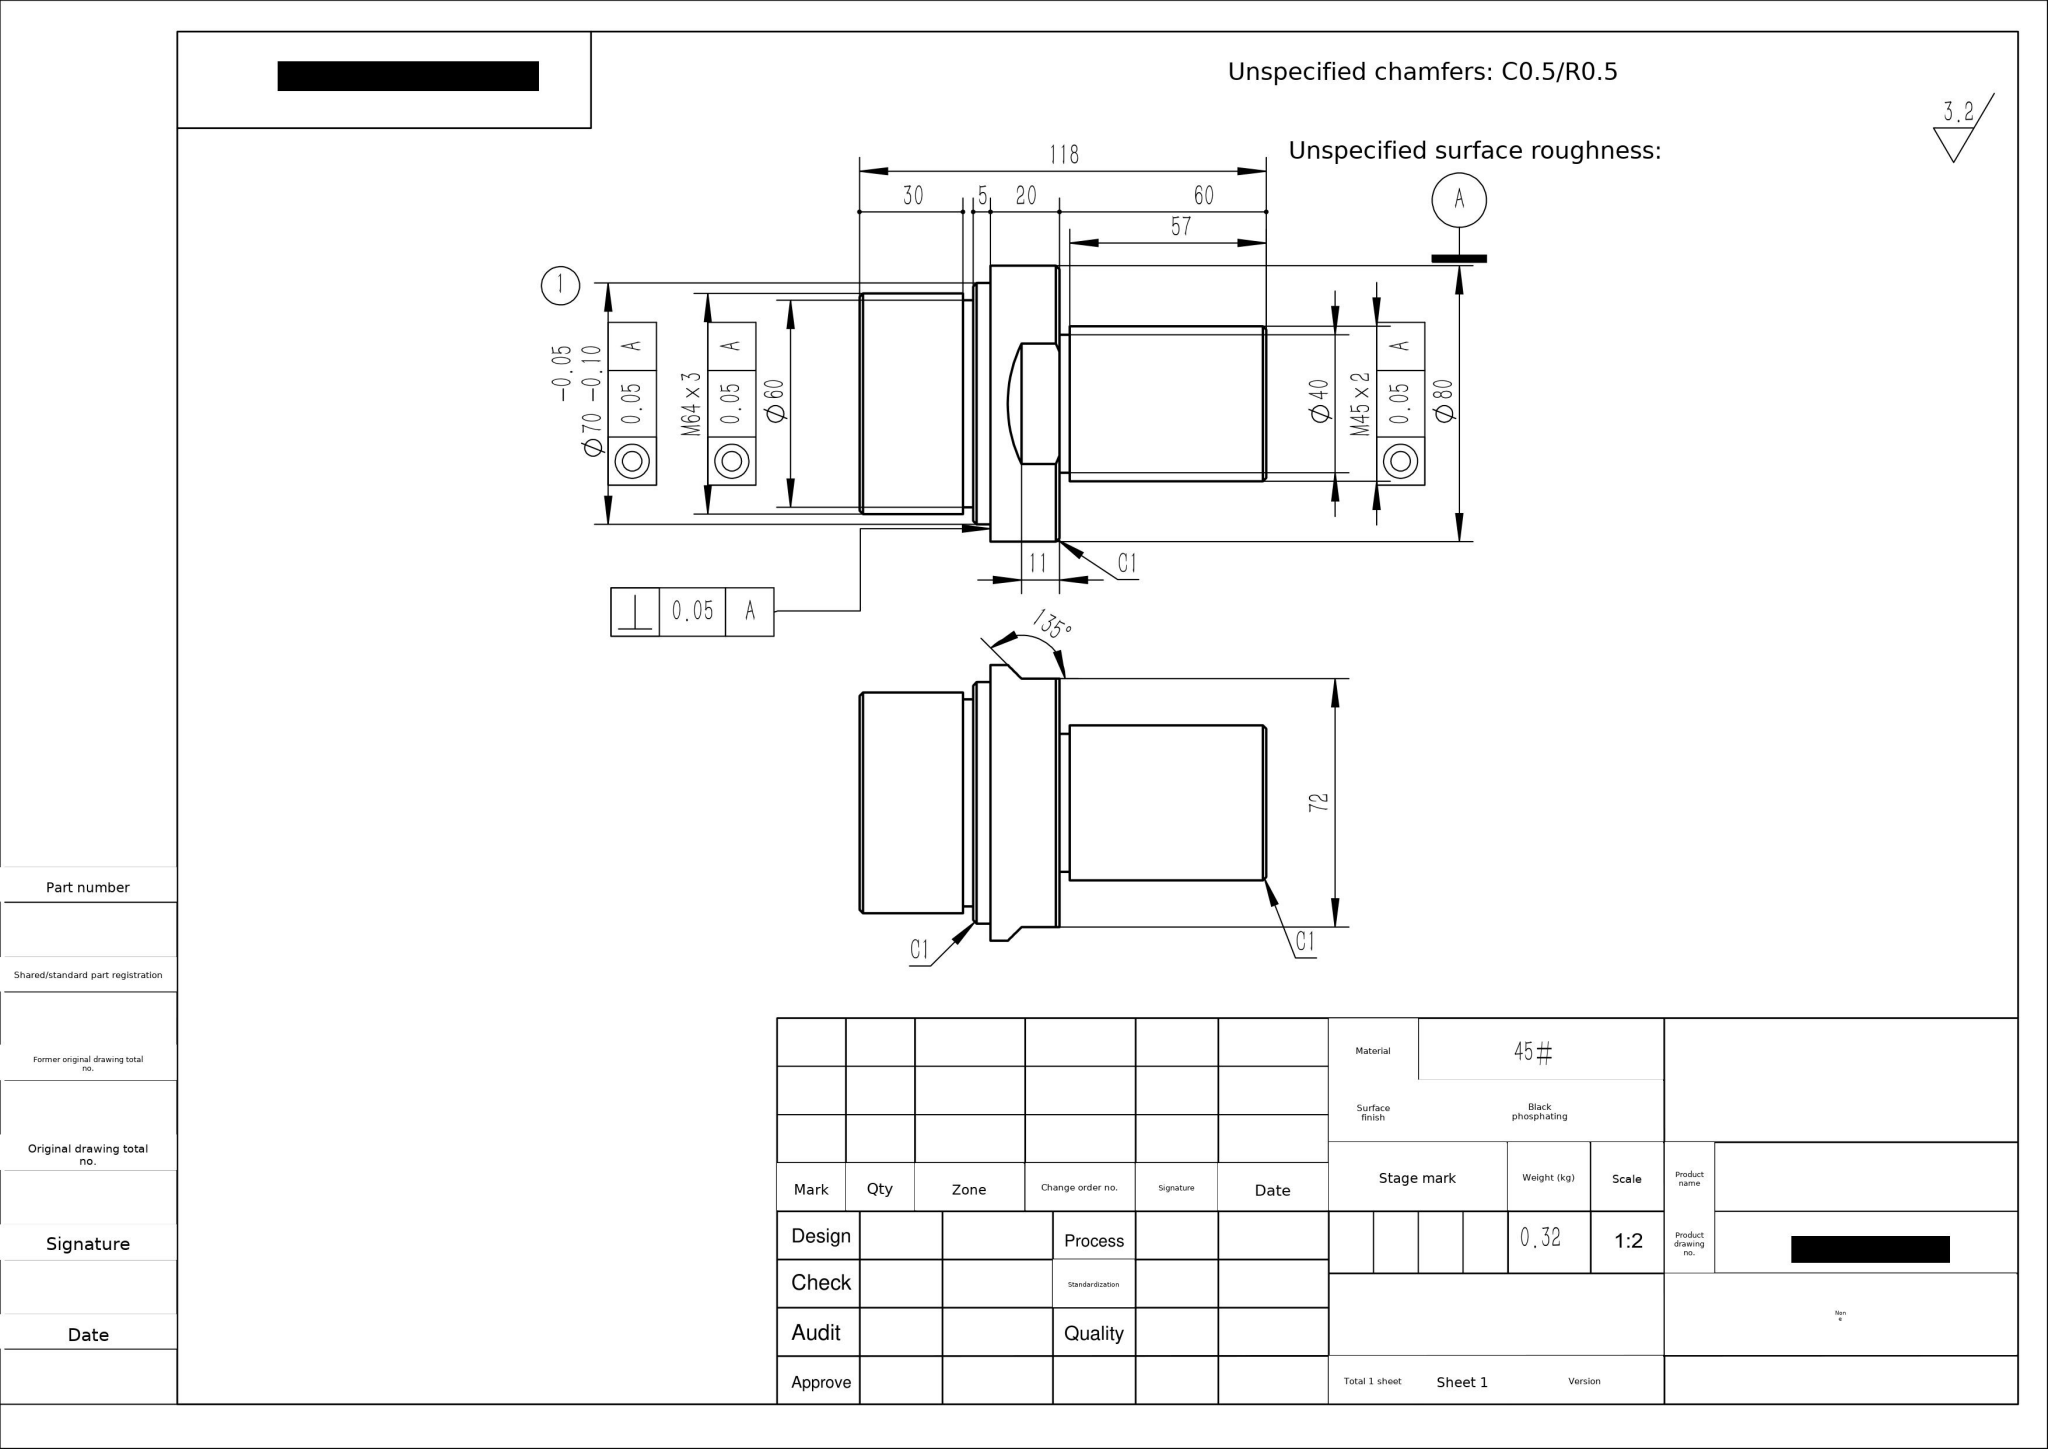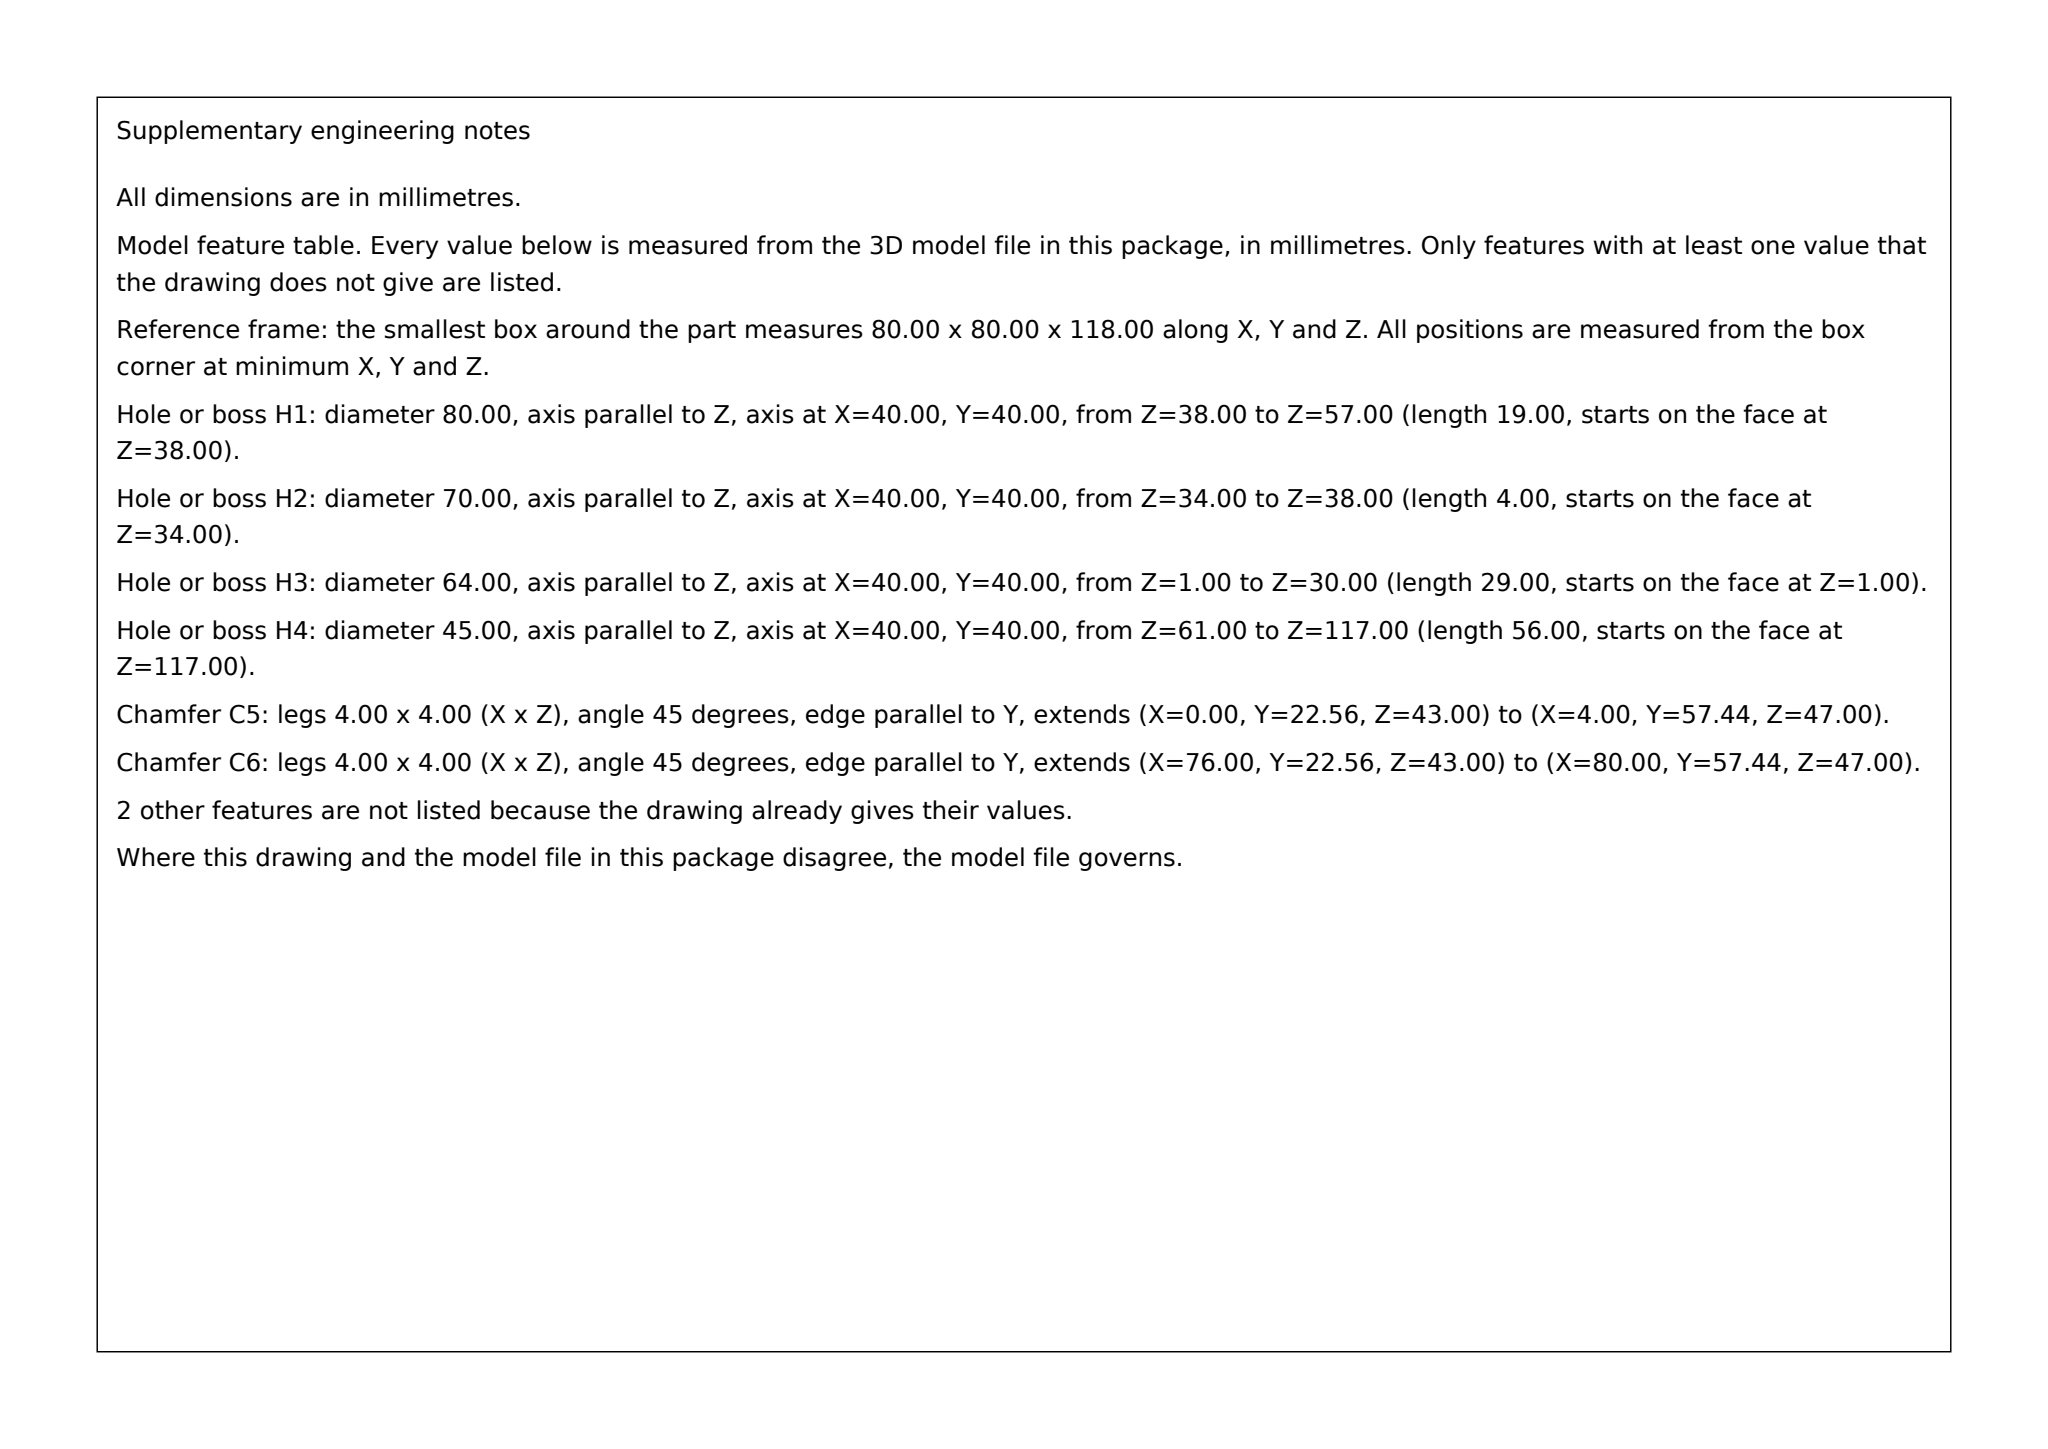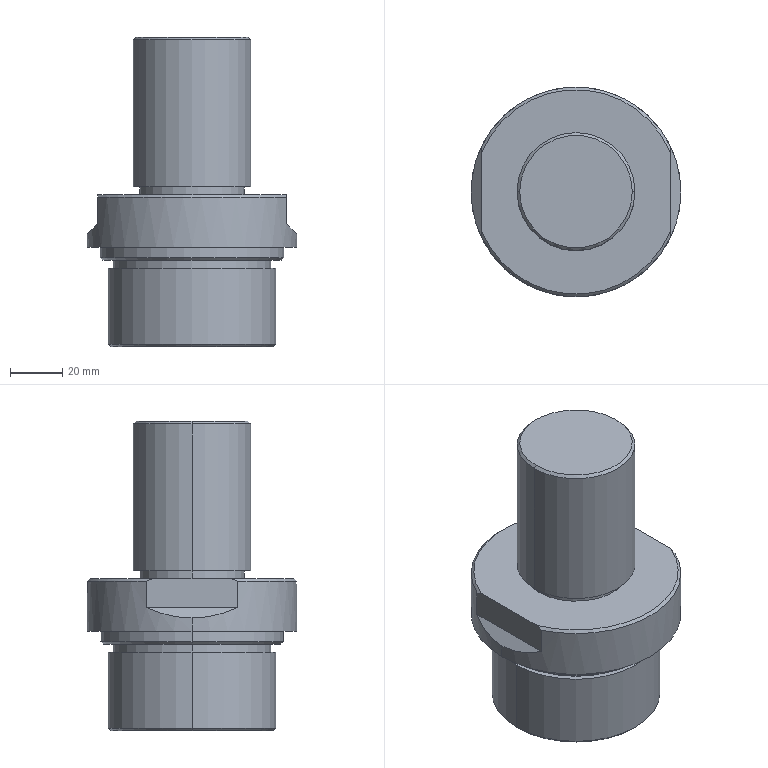Part | SolidWorks | mm | material 45# | 1 solid | 31 faces | box 80 x 80 x 118 mm | volume 316452 mm3 | cylinder 12 | plane 11 | cone 8 | commonest cylinder face diameters 45 x2 40 x2 80 x2 70 x2 60 x2 64 x2
STEP:
#1=CARTESIAN_POINT('',(21.5,0.,118.));
#2=VERTEX_POINT('',#1);
#3=CARTESIAN_POINT('',(-21.5,0.,118.));
#4=VERTEX_POINT('',#3);
#5=CARTESIAN_POINT('',(0.,0.,118.));
#6=DIRECTION('',(0.,0.,1.));
#7=DIRECTION('',(1.,0.,0.));
#8=AXIS2_PLACEMENT_3D('',#5,#6,#7);
#9=CIRCLE('',#8,21.5);
#10=EDGE_CURVE('',#2,#4,#9,.T.);
#11=ORIENTED_EDGE('',*,*,#10,.F.);
#12=CARTESIAN_POINT('',(22.5,0.,117.));
#13=VERTEX_POINT('',#12);
#14=CARTESIAN_POINT('',(21.5,0.,118.));
#15=DIRECTION('',(0.7071,0.,-0.7071));
#16=VECTOR('',#15,1000.);
#17=LINE('',#14,#16);
#18=EDGE_CURVE('',#2,#13,#17,.T.);
#19=ORIENTED_EDGE('',*,*,#18,.T.);
#20=CARTESIAN_POINT('',(-22.5,0.,117.));
#21=VERTEX_POINT('',#20);
#22=CARTESIAN_POINT('',(0.,0.,117.));
#23=DIRECTION('',(0.,0.,-1.));
#24=DIRECTION('',(1.,0.,0.));
#25=AXIS2_PLACEMENT_3D('',#22,#23,#24);
#26=CIRCLE('',#25,22.5);
#27=EDGE_CURVE('',#21,#13,#26,.T.);
#28=ORIENTED_EDGE('',*,*,#27,.F.);
#29=CARTESIAN_POINT('',(-21.5,0.,118.));
#30=DIRECTION('',(-0.7071,0.,-0.7071));
#31=VECTOR('',#30,1000.);
#32=LINE('',#29,#31);
#33=EDGE_CURVE('',#4,#21,#32,.T.);
#34=ORIENTED_EDGE('',*,*,#33,.F.);
#35=EDGE_LOOP('',(#11,#19,#28,#34));
#36=FACE_OUTER_BOUND('',#35,.T.);
#37=CARTESIAN_POINT('',(0.,0.,118.));
#38=DIRECTION('',(0.,0.,-1.));
#39=DIRECTION('',(-1.,0.,0.));
#40=AXIS2_PLACEMENT_3D('',#37,#38,#39);
#41=CONICAL_SURFACE('',#40,21.5,0.7854);
#42=ADVANCED_FACE('',(#36),#41,.T.);
#43=CARTESIAN_POINT('',(-34.,0.,33.));
#44=VERTEX_POINT('',#43);
#45=CARTESIAN_POINT('',(34.,0.,33.));
#46=VERTEX_POINT('',#45);
#47=CARTESIAN_POINT('',(0.,0.,33.));
#48=DIRECTION('',(0.,0.,-1.));
#49=DIRECTION('',(1.,0.,0.));
#50=AXIS2_PLACEMENT_3D('',#47,#48,#49);
#51=CIRCLE('',#50,34.);
#52=EDGE_CURVE('',#44,#46,#51,.T.);
#53=ORIENTED_EDGE('',*,*,#52,.F.);
#54=CARTESIAN_POINT('',(-35.,0.,34.));
#55=VERTEX_POINT('',#54);
#56=CARTESIAN_POINT('',(-35.,0.,34.));
#57=DIRECTION('',(-0.7071,0.,0.7071));
#58=VECTOR('',#57,1000.);
#59=LINE('',#56,#58);
#60=EDGE_CURVE('',#44,#55,#59,.T.);
#61=ORIENTED_EDGE('',*,*,#60,.T.);
#62=CARTESIAN_POINT('',(35.,0.,34.));
#63=VERTEX_POINT('',#62);
#64=CARTESIAN_POINT('',(0.,0.,34.));
#65=DIRECTION('',(0.,0.,1.));
#66=DIRECTION('',(1.,0.,0.));
#67=AXIS2_PLACEMENT_3D('',#64,#65,#66);
#68=CIRCLE('',#67,35.);
#69=EDGE_CURVE('',#63,#55,#68,.T.);
#70=ORIENTED_EDGE('',*,*,#69,.F.);
#71=CARTESIAN_POINT('',(35.,0.,34.));
#72=DIRECTION('',(0.7071,0.,0.7071));
#73=VECTOR('',#72,1000.);
#74=LINE('',#71,#73);
#75=EDGE_CURVE('',#46,#63,#74,.T.);
#76=ORIENTED_EDGE('',*,*,#75,.F.);
#77=EDGE_LOOP('',(#53,#61,#70,#76));
#78=FACE_OUTER_BOUND('',#77,.T.);
#79=CARTESIAN_POINT('',(0.,0.,34.));
#80=DIRECTION('',(0.,0.,1.));
#81=DIRECTION('',(1.,0.,0.));
#82=AXIS2_PLACEMENT_3D('',#79,#80,#81);
#83=CONICAL_SURFACE('',#82,35.,0.7854);
#84=ADVANCED_FACE('',(#78),#83,.T.);
#85=CARTESIAN_POINT('',(-31.,0.,0.));
#86=VERTEX_POINT('',#85);
#87=CARTESIAN_POINT('',(31.,0.,0.));
#88=VERTEX_POINT('',#87);
#89=CARTESIAN_POINT('',(0.,0.,0.));
#90=DIRECTION('',(0.,0.,-1.));
#91=DIRECTION('',(1.,0.,0.));
#92=AXIS2_PLACEMENT_3D('',#89,#90,#91);
#93=CIRCLE('',#92,31.);
#94=EDGE_CURVE('',#86,#88,#93,.T.);
#95=ORIENTED_EDGE('',*,*,#94,.F.);
#96=CARTESIAN_POINT('',(-32.,0.,1.));
#97=VERTEX_POINT('',#96);
#98=CARTESIAN_POINT('',(-32.,0.,1.));
#99=DIRECTION('',(-0.7071,0.,0.7071));
#100=VECTOR('',#99,1000.);
#101=LINE('',#98,#100);
#102=EDGE_CURVE('',#86,#97,#101,.T.);
#103=ORIENTED_EDGE('',*,*,#102,.T.);
#104=CARTESIAN_POINT('',(32.,0.,1.));
#105=VERTEX_POINT('',#104);
#106=CARTESIAN_POINT('',(0.,0.,1.));
#107=DIRECTION('',(0.,0.,1.));
#108=DIRECTION('',(1.,0.,0.));
#109=AXIS2_PLACEMENT_3D('',#106,#107,#108);
#110=CIRCLE('',#109,32.);
#111=EDGE_CURVE('',#105,#97,#110,.T.);
#112=ORIENTED_EDGE('',*,*,#111,.F.);
#113=CARTESIAN_POINT('',(32.,0.,1.));
#114=DIRECTION('',(0.7071,0.,0.7071));
#115=VECTOR('',#114,1000.);
#116=LINE('',#113,#115);
#117=EDGE_CURVE('',#88,#105,#116,.T.);
#118=ORIENTED_EDGE('',*,*,#117,.F.);
#119=EDGE_LOOP('',(#95,#103,#112,#118));
#120=FACE_OUTER_BOUND('',#119,.T.);
#121=CARTESIAN_POINT('',(0.,0.,1.));
#122=DIRECTION('',(0.,0.,1.));
#123=DIRECTION('',(1.,0.,0.));
#124=AXIS2_PLACEMENT_3D('',#121,#122,#123);
#125=CONICAL_SURFACE('',#124,32.,0.7854);
#126=ADVANCED_FACE('',(#120),#125,.T.);
#127=ORIENTED_EDGE('',*,*,#27,.T.);
#128=CARTESIAN_POINT('',(22.5,0.,61.));
#129=VERTEX_POINT('',#128);
#130=CARTESIAN_POINT('',(22.5,0.,118.));
#131=DIRECTION('',(0.,0.,-1.));
#132=VECTOR('',#131,1000.);
#133=LINE('',#130,#132);
#134=EDGE_CURVE('',#13,#129,#133,.T.);
#135=ORIENTED_EDGE('',*,*,#134,.T.);
#136=CARTESIAN_POINT('',(-22.5,0.,61.));
#137=VERTEX_POINT('',#136);
#138=CARTESIAN_POINT('',(0.,0.,61.));
#139=DIRECTION('',(0.,0.,1.));
#140=DIRECTION('',(1.,0.,0.));
#141=AXIS2_PLACEMENT_3D('',#138,#139,#140);
#142=CIRCLE('',#141,22.5);
#143=EDGE_CURVE('',#129,#137,#142,.T.);
#144=ORIENTED_EDGE('',*,*,#143,.T.);
#145=CARTESIAN_POINT('',(-22.5,0.,118.));
#146=DIRECTION('',(0.,0.,-1.));
#147=VECTOR('',#146,1000.);
#148=LINE('',#145,#147);
#149=EDGE_CURVE('',#21,#137,#148,.T.);
#150=ORIENTED_EDGE('',*,*,#149,.F.);
#151=EDGE_LOOP('',(#127,#135,#144,#150));
#152=FACE_OUTER_BOUND('',#151,.T.);
#153=CARTESIAN_POINT('',(0.,0.,118.));
#154=DIRECTION('',(0.,0.,-1.));
#155=DIRECTION('',(-1.,0.,0.));
#156=AXIS2_PLACEMENT_3D('',#153,#154,#155);
#157=CYLINDRICAL_SURFACE('',#156,22.5);
#158=ADVANCED_FACE('',(#152),#157,.T.);
#159=CARTESIAN_POINT('',(20.,0.,61.));
#160=VERTEX_POINT('',#159);
#161=CARTESIAN_POINT('',(-20.,0.,61.));
#162=VERTEX_POINT('',#161);
#163=CARTESIAN_POINT('',(0.,0.,61.));
#164=DIRECTION('',(0.,0.,1.));
#165=DIRECTION('',(1.,0.,0.));
#166=AXIS2_PLACEMENT_3D('',#163,#164,#165);
#167=CIRCLE('',#166,20.);
#168=EDGE_CURVE('',#160,#162,#167,.T.);
#169=ORIENTED_EDGE('',*,*,#168,.F.);
#170=CARTESIAN_POINT('',(20.,0.,58.));
#171=VERTEX_POINT('',#170);
#172=CARTESIAN_POINT('',(20.,0.,61.));
#173=DIRECTION('',(0.,0.,-1.));
#174=VECTOR('',#173,1000.);
#175=LINE('',#172,#174);
#176=EDGE_CURVE('',#160,#171,#175,.T.);
#177=ORIENTED_EDGE('',*,*,#176,.T.);
#178=CARTESIAN_POINT('',(-20.,0.,58.));
#179=VERTEX_POINT('',#178);
#180=CARTESIAN_POINT('',(0.,0.,58.));
#181=DIRECTION('',(0.,0.,1.));
#182=DIRECTION('',(1.,0.,0.));
#183=AXIS2_PLACEMENT_3D('',#180,#181,#182);
#184=CIRCLE('',#183,20.);
#185=EDGE_CURVE('',#171,#179,#184,.T.);
#186=ORIENTED_EDGE('',*,*,#185,.T.);
#187=CARTESIAN_POINT('',(-20.,0.,61.));
#188=DIRECTION('',(0.,0.,-1.));
#189=VECTOR('',#188,1000.);
#190=LINE('',#187,#189);
#191=EDGE_CURVE('',#162,#179,#190,.T.);
#192=ORIENTED_EDGE('',*,*,#191,.F.);
#193=EDGE_LOOP('',(#169,#177,#186,#192));
#194=FACE_OUTER_BOUND('',#193,.T.);
#195=CARTESIAN_POINT('',(0.,0.,61.));
#196=DIRECTION('',(0.,0.,-1.));
#197=DIRECTION('',(-1.,0.,0.));
#198=AXIS2_PLACEMENT_3D('',#195,#196,#197);
#199=CYLINDRICAL_SURFACE('',#198,20.);
#200=ADVANCED_FACE('',(#194),#199,.T.);
#201=CARTESIAN_POINT('',(36.,17.436,47.));
#202=VERTEX_POINT('',#201);
#203=CARTESIAN_POINT('',(40.,0.,43.));
#204=VERTEX_POINT('',#203);
#205=CARTESIAN_POINT('',(36.,17.436,47.));
#206=CARTESIAN_POINT('',(38.644,11.977,44.356));
#207=CARTESIAN_POINT('',(40.,6.065,43.));
#208=CARTESIAN_POINT('',(40.,0.,43.));
#209=(BOUNDED_CURVE()B_SPLINE_CURVE(3,(#205,#206,#207,#208),.UNSPECIFIED.,.F.,.T.)B_SPLINE_CURVE_WITH_KNOTS((4,4),(5.832,6.283),.UNSPECIFIED.)CURVE()GEOMETRIC_REPRESENTATION_ITEM()RATIONAL_B_SPLINE_CURVE((1.,0.9831,0.9831,1.))REPRESENTATION_ITEM(''));
#210=EDGE_CURVE('',#202,#204,#209,.T.);
#211=ORIENTED_EDGE('',*,*,#210,.T.);
#212=CARTESIAN_POINT('',(40.,0.,38.));
#213=VERTEX_POINT('',#212);
#214=CARTESIAN_POINT('',(40.,0.,58.));
#215=DIRECTION('',(0.,0.,-1.));
#216=VECTOR('',#215,1000.);
#217=LINE('',#214,#216);
#218=EDGE_CURVE('',#204,#213,#217,.T.);
#219=ORIENTED_EDGE('',*,*,#218,.T.);
#220=CARTESIAN_POINT('',(-40.,0.,38.));
#221=VERTEX_POINT('',#220);
#222=CARTESIAN_POINT('',(0.,0.,38.));
#223=DIRECTION('',(0.,0.,1.));
#224=DIRECTION('',(1.,0.,0.));
#225=AXIS2_PLACEMENT_3D('',#222,#223,#224);
#226=CIRCLE('',#225,40.);
#227=EDGE_CURVE('',#213,#221,#226,.T.);
#228=ORIENTED_EDGE('',*,*,#227,.T.);
#229=CARTESIAN_POINT('',(-40.,0.,43.));
#230=VERTEX_POINT('',#229);
#231=CARTESIAN_POINT('',(-40.,0.,58.));
#232=DIRECTION('',(0.,0.,-1.));
#233=VECTOR('',#232,1000.);
#234=LINE('',#231,#233);
#235=EDGE_CURVE('',#230,#221,#234,.T.);
#236=ORIENTED_EDGE('',*,*,#235,.F.);
#237=CARTESIAN_POINT('',(-36.,17.436,47.));
#238=VERTEX_POINT('',#237);
#239=CARTESIAN_POINT('',(-40.,0.,43.));
#240=CARTESIAN_POINT('',(-40.,6.065,43.));
#241=CARTESIAN_POINT('',(-38.644,11.977,44.356));
#242=CARTESIAN_POINT('',(-36.,17.436,47.));
#243=(BOUNDED_CURVE()B_SPLINE_CURVE(3,(#239,#240,#241,#242),.UNSPECIFIED.,.F.,.T.)B_SPLINE_CURVE_WITH_KNOTS((4,4),(0.,0.451),.UNSPECIFIED.)CURVE()GEOMETRIC_REPRESENTATION_ITEM()RATIONAL_B_SPLINE_CURVE((1.,0.9831,0.9831,1.))REPRESENTATION_ITEM(''));
#244=EDGE_CURVE('',#230,#238,#243,.T.);
#245=ORIENTED_EDGE('',*,*,#244,.T.);
#246=CARTESIAN_POINT('',(-36.,17.436,57.));
#247=VERTEX_POINT('',#246);
#248=CARTESIAN_POINT('',(-36.,17.436,58.));
#249=DIRECTION('',(0.,0.,1.));
#250=VECTOR('',#249,1000.);
#251=LINE('',#248,#250);
#252=EDGE_CURVE('',#238,#247,#251,.T.);
#253=ORIENTED_EDGE('',*,*,#252,.T.);
#254=CARTESIAN_POINT('',(36.,17.436,57.));
#255=VERTEX_POINT('',#254);
#256=CARTESIAN_POINT('',(0.,0.,57.));
#257=DIRECTION('',(0.,0.,-1.));
#258=DIRECTION('',(1.,0.,0.));
#259=AXIS2_PLACEMENT_3D('',#256,#257,#258);
#260=CIRCLE('',#259,40.);
#261=EDGE_CURVE('',#247,#255,#260,.T.);
#262=ORIENTED_EDGE('',*,*,#261,.T.);
#263=CARTESIAN_POINT('',(36.,17.436,58.));
#264=DIRECTION('',(0.,0.,-1.));
#265=VECTOR('',#264,1000.);
#266=LINE('',#263,#265);
#267=EDGE_CURVE('',#255,#202,#266,.T.);
#268=ORIENTED_EDGE('',*,*,#267,.T.);
#269=EDGE_LOOP('',(#211,#219,#228,#236,#245,#253,#262,#268));
#270=FACE_OUTER_BOUND('',#269,.T.);
#271=CARTESIAN_POINT('',(0.,0.,58.));
#272=DIRECTION('',(0.,0.,-1.));
#273=DIRECTION('',(-1.,0.,0.));
#274=AXIS2_PLACEMENT_3D('',#271,#272,#273);
#275=CYLINDRICAL_SURFACE('',#274,40.);
#276=ADVANCED_FACE('',(#270),#275,.T.);
#277=CARTESIAN_POINT('',(35.,0.,38.));
#278=VERTEX_POINT('',#277);
#279=CARTESIAN_POINT('',(-35.,0.,38.));
#280=VERTEX_POINT('',#279);
#281=CARTESIAN_POINT('',(0.,0.,38.));
#282=DIRECTION('',(0.,0.,1.));
#283=DIRECTION('',(1.,0.,0.));
#284=AXIS2_PLACEMENT_3D('',#281,#282,#283);
#285=CIRCLE('',#284,35.);
#286=EDGE_CURVE('',#278,#280,#285,.T.);
#287=ORIENTED_EDGE('',*,*,#286,.F.);
#288=CARTESIAN_POINT('',(35.,0.,38.));
#289=DIRECTION('',(0.,0.,-1.));
#290=VECTOR('',#289,1000.);
#291=LINE('',#288,#290);
#292=EDGE_CURVE('',#278,#63,#291,.T.);
#293=ORIENTED_EDGE('',*,*,#292,.T.);
#294=ORIENTED_EDGE('',*,*,#69,.T.);
#295=CARTESIAN_POINT('',(-35.,0.,38.));
#296=DIRECTION('',(0.,0.,-1.));
#297=VECTOR('',#296,1000.);
#298=LINE('',#295,#297);
#299=EDGE_CURVE('',#280,#55,#298,.T.);
#300=ORIENTED_EDGE('',*,*,#299,.F.);
#301=EDGE_LOOP('',(#287,#293,#294,#300));
#302=FACE_OUTER_BOUND('',#301,.T.);
#303=CARTESIAN_POINT('',(0.,0.,38.));
#304=DIRECTION('',(0.,0.,-1.));
#305=DIRECTION('',(-1.,0.,0.));
#306=AXIS2_PLACEMENT_3D('',#303,#304,#305);
#307=CYLINDRICAL_SURFACE('',#306,35.);
#308=ADVANCED_FACE('',(#302),#307,.T.);
#309=CARTESIAN_POINT('',(30.,0.,33.));
#310=VERTEX_POINT('',#309);
#311=CARTESIAN_POINT('',(-30.,0.,33.));
#312=VERTEX_POINT('',#311);
#313=CARTESIAN_POINT('',(0.,0.,33.));
#314=DIRECTION('',(0.,0.,1.));
#315=DIRECTION('',(1.,0.,0.));
#316=AXIS2_PLACEMENT_3D('',#313,#314,#315);
#317=CIRCLE('',#316,30.);
#318=EDGE_CURVE('',#310,#312,#317,.T.);
#319=ORIENTED_EDGE('',*,*,#318,.F.);
#320=CARTESIAN_POINT('',(30.,0.,30.));
#321=VERTEX_POINT('',#320);
#322=CARTESIAN_POINT('',(30.,0.,33.));
#323=DIRECTION('',(0.,0.,-1.));
#324=VECTOR('',#323,1000.);
#325=LINE('',#322,#324);
#326=EDGE_CURVE('',#310,#321,#325,.T.);
#327=ORIENTED_EDGE('',*,*,#326,.T.);
#328=CARTESIAN_POINT('',(-30.,0.,30.));
#329=VERTEX_POINT('',#328);
#330=CARTESIAN_POINT('',(0.,0.,30.));
#331=DIRECTION('',(0.,0.,1.));
#332=DIRECTION('',(1.,0.,0.));
#333=AXIS2_PLACEMENT_3D('',#330,#331,#332);
#334=CIRCLE('',#333,30.);
#335=EDGE_CURVE('',#321,#329,#334,.T.);
#336=ORIENTED_EDGE('',*,*,#335,.T.);
#337=CARTESIAN_POINT('',(-30.,0.,33.));
#338=DIRECTION('',(0.,0.,-1.));
#339=VECTOR('',#338,1000.);
#340=LINE('',#337,#339);
#341=EDGE_CURVE('',#312,#329,#340,.T.);
#342=ORIENTED_EDGE('',*,*,#341,.F.);
#343=EDGE_LOOP('',(#319,#327,#336,#342));
#344=FACE_OUTER_BOUND('',#343,.T.);
#345=CARTESIAN_POINT('',(0.,0.,33.));
#346=DIRECTION('',(0.,0.,-1.));
#347=DIRECTION('',(-1.,0.,0.));
#348=AXIS2_PLACEMENT_3D('',#345,#346,#347);
#349=CYLINDRICAL_SURFACE('',#348,30.);
#350=ADVANCED_FACE('',(#344),#349,.T.);
#351=CARTESIAN_POINT('',(32.,0.,30.));
#352=VERTEX_POINT('',#351);
#353=CARTESIAN_POINT('',(-32.,0.,30.));
#354=VERTEX_POINT('',#353);
#355=CARTESIAN_POINT('',(0.,0.,30.));
#356=DIRECTION('',(0.,0.,1.));
#357=DIRECTION('',(1.,0.,0.));
#358=AXIS2_PLACEMENT_3D('',#355,#356,#357);
#359=CIRCLE('',#358,32.);
#360=EDGE_CURVE('',#352,#354,#359,.T.);
#361=ORIENTED_EDGE('',*,*,#360,.F.);
#362=CARTESIAN_POINT('',(32.,0.,30.));
#363=DIRECTION('',(0.,0.,-1.));
#364=VECTOR('',#363,1000.);
#365=LINE('',#362,#364);
#366=EDGE_CURVE('',#352,#105,#365,.T.);
#367=ORIENTED_EDGE('',*,*,#366,.T.);
#368=ORIENTED_EDGE('',*,*,#111,.T.);
#369=CARTESIAN_POINT('',(-32.,0.,30.));
#370=DIRECTION('',(0.,0.,-1.));
#371=VECTOR('',#370,1000.);
#372=LINE('',#369,#371);
#373=EDGE_CURVE('',#354,#97,#372,.T.);
#374=ORIENTED_EDGE('',*,*,#373,.F.);
#375=EDGE_LOOP('',(#361,#367,#368,#374));
#376=FACE_OUTER_BOUND('',#375,.T.);
#377=CARTESIAN_POINT('',(0.,0.,30.));
#378=DIRECTION('',(0.,0.,-1.));
#379=DIRECTION('',(-1.,0.,0.));
#380=AXIS2_PLACEMENT_3D('',#377,#378,#379);
#381=CYLINDRICAL_SURFACE('',#380,32.);
#382=ADVANCED_FACE('',(#376),#381,.T.);
#383=CARTESIAN_POINT('',(-36.,-17.436,57.));
#384=VERTEX_POINT('',#383);
#385=CARTESIAN_POINT('',(-36.,-15.,58.));
#386=VERTEX_POINT('',#385);
#387=CARTESIAN_POINT('',(-36.,-17.436,57.));
#388=CARTESIAN_POINT('',(-36.,-16.631,57.351));
#389=CARTESIAN_POINT('',(-36.,-15.82,57.685));
#390=CARTESIAN_POINT('',(-36.,-15.,58.));
#391=B_SPLINE_CURVE_WITH_KNOTS('',3,(#387,#388,#389,#390),.UNSPECIFIED.,.F.,.F.,(4,4),(0.07863,0.08127),.UNSPECIFIED.);
#392=EDGE_CURVE('',#384,#386,#391,.T.);
#393=ORIENTED_EDGE('',*,*,#392,.F.);
#394=CARTESIAN_POINT('',(36.,-17.436,57.));
#395=VERTEX_POINT('',#394);
#396=CARTESIAN_POINT('',(0.,0.,57.));
#397=DIRECTION('',(0.,0.,-1.));
#398=DIRECTION('',(1.,0.,0.));
#399=AXIS2_PLACEMENT_3D('',#396,#397,#398);
#400=CIRCLE('',#399,40.);
#401=EDGE_CURVE('',#395,#384,#400,.T.);
#402=ORIENTED_EDGE('',*,*,#401,.F.);
#403=CARTESIAN_POINT('',(36.,-15.,58.));
#404=VERTEX_POINT('',#403);
#405=CARTESIAN_POINT('',(36.,-15.,58.));
#406=CARTESIAN_POINT('',(36.,-15.822,57.684));
#407=CARTESIAN_POINT('',(36.,-16.634,57.35));
#408=CARTESIAN_POINT('',(36.,-17.436,57.));
#409=B_SPLINE_CURVE_WITH_KNOTS('',3,(#405,#406,#407,#408),.UNSPECIFIED.,.F.,.F.,(4,4),(0.112,0.1146),.UNSPECIFIED.);
#410=EDGE_CURVE('',#404,#395,#409,.T.);
#411=ORIENTED_EDGE('',*,*,#410,.F.);
#412=CARTESIAN_POINT('',(0.,0.,58.));
#413=DIRECTION('',(0.,0.,1.));
#414=DIRECTION('',(1.,0.,0.));
#415=AXIS2_PLACEMENT_3D('',#412,#413,#414);
#416=CIRCLE('',#415,39.);
#417=EDGE_CURVE('',#386,#404,#416,.T.);
#418=ORIENTED_EDGE('',*,*,#417,.F.);
#419=EDGE_LOOP('',(#393,#402,#411,#418));
#420=FACE_OUTER_BOUND('',#419,.T.);
#421=CARTESIAN_POINT('',(0.,0.,58.));
#422=DIRECTION('',(0.,0.,-1.));
#423=DIRECTION('',(-1.,0.,0.));
#424=AXIS2_PLACEMENT_3D('',#421,#422,#423);
#425=CONICAL_SURFACE('',#424,39.,0.7854);
#426=ADVANCED_FACE('',(#420),#425,.T.);
#427=ORIENTED_EDGE('',*,*,#366,.F.);
#428=CARTESIAN_POINT('',(0.,0.,30.));
#429=DIRECTION('',(0.,0.,1.));
#430=DIRECTION('',(1.,0.,0.));
#431=AXIS2_PLACEMENT_3D('',#428,#429,#430);
#432=CIRCLE('',#431,32.);
#433=EDGE_CURVE('',#354,#352,#432,.T.);
#434=ORIENTED_EDGE('',*,*,#433,.F.);
#435=ORIENTED_EDGE('',*,*,#373,.T.);
#436=CARTESIAN_POINT('',(0.,0.,1.));
#437=DIRECTION('',(0.,0.,1.));
#438=DIRECTION('',(1.,0.,0.));
#439=AXIS2_PLACEMENT_3D('',#436,#437,#438);
#440=CIRCLE('',#439,32.);
#441=EDGE_CURVE('',#97,#105,#440,.T.);
#442=ORIENTED_EDGE('',*,*,#441,.T.);
#443=EDGE_LOOP('',(#427,#434,#435,#442));
#444=FACE_OUTER_BOUND('',#443,.T.);
#445=CARTESIAN_POINT('',(0.,0.,30.));
#446=DIRECTION('',(0.,0.,-1.));
#447=DIRECTION('',(-1.,0.,0.));
#448=AXIS2_PLACEMENT_3D('',#445,#446,#447);
#449=CYLINDRICAL_SURFACE('',#448,32.);
#450=ADVANCED_FACE('',(#444),#449,.T.);
#451=CARTESIAN_POINT('',(0.,0.,30.));
#452=DIRECTION('',(0.,0.,1.));
#453=DIRECTION('',(1.,0.,0.));
#454=AXIS2_PLACEMENT_3D('',#451,#452,#453);
#455=CIRCLE('',#454,30.);
#456=EDGE_CURVE('',#329,#321,#455,.T.);
#457=ORIENTED_EDGE('',*,*,#456,.F.);
#458=ORIENTED_EDGE('',*,*,#335,.F.);
#459=EDGE_LOOP('',(#457,#458));
#460=FACE_BOUND('',#459,.T.);
#461=ORIENTED_EDGE('',*,*,#433,.T.);
#462=ORIENTED_EDGE('',*,*,#360,.T.);
#463=EDGE_LOOP('',(#461,#462));
#464=FACE_OUTER_BOUND('',#463,.T.);
#465=CARTESIAN_POINT('',(0.,0.,30.));
#466=DIRECTION('',(0.,0.,1.));
#467=DIRECTION('',(1.,0.,0.));
#468=AXIS2_PLACEMENT_3D('',#465,#466,#467);
#469=PLANE('',#468);
#470=ADVANCED_FACE('',(#460,#464),#469,.T.);
#471=CARTESIAN_POINT('',(0.,0.,0.));
#472=DIRECTION('',(0.,0.,-1.));
#473=DIRECTION('',(1.,0.,0.));
#474=AXIS2_PLACEMENT_3D('',#471,#472,#473);
#475=CIRCLE('',#474,31.);
#476=EDGE_CURVE('',#88,#86,#475,.T.);
#477=ORIENTED_EDGE('',*,*,#476,.T.);
#478=ORIENTED_EDGE('',*,*,#94,.T.);
#479=EDGE_LOOP('',(#477,#478));
#480=FACE_OUTER_BOUND('',#479,.T.);
#481=CARTESIAN_POINT('',(0.,0.,0.));
#482=DIRECTION('',(0.,0.,1.));
#483=DIRECTION('',(1.,0.,0.));
#484=AXIS2_PLACEMENT_3D('',#481,#482,#483);
#485=PLANE('',#484);
#486=ADVANCED_FACE('',(#480),#485,.F.);
#487=ORIENTED_EDGE('',*,*,#326,.F.);
#488=CARTESIAN_POINT('',(0.,0.,33.));
#489=DIRECTION('',(0.,0.,1.));
#490=DIRECTION('',(1.,0.,0.));
#491=AXIS2_PLACEMENT_3D('',#488,#489,#490);
#492=CIRCLE('',#491,30.);
#493=EDGE_CURVE('',#312,#310,#492,.T.);
#494=ORIENTED_EDGE('',*,*,#493,.F.);
#495=ORIENTED_EDGE('',*,*,#341,.T.);
#496=ORIENTED_EDGE('',*,*,#456,.T.);
#497=EDGE_LOOP('',(#487,#494,#495,#496));
#498=FACE_OUTER_BOUND('',#497,.T.);
#499=CARTESIAN_POINT('',(0.,0.,33.));
#500=DIRECTION('',(0.,0.,-1.));
#501=DIRECTION('',(-1.,0.,0.));
#502=AXIS2_PLACEMENT_3D('',#499,#500,#501);
#503=CYLINDRICAL_SURFACE('',#502,30.);
#504=ADVANCED_FACE('',(#498),#503,.T.);
#505=ORIENTED_EDGE('',*,*,#292,.F.);
#506=CARTESIAN_POINT('',(0.,0.,38.));
#507=DIRECTION('',(0.,0.,1.));
#508=DIRECTION('',(1.,0.,0.));
#509=AXIS2_PLACEMENT_3D('',#506,#507,#508);
#510=CIRCLE('',#509,35.);
#511=EDGE_CURVE('',#280,#278,#510,.T.);
#512=ORIENTED_EDGE('',*,*,#511,.F.);
#513=ORIENTED_EDGE('',*,*,#299,.T.);
#514=CARTESIAN_POINT('',(0.,0.,34.));
#515=DIRECTION('',(0.,0.,1.));
#516=DIRECTION('',(1.,0.,0.));
#517=AXIS2_PLACEMENT_3D('',#514,#515,#516);
#518=CIRCLE('',#517,35.);
#519=EDGE_CURVE('',#55,#63,#518,.T.);
#520=ORIENTED_EDGE('',*,*,#519,.T.);
#521=EDGE_LOOP('',(#505,#512,#513,#520));
#522=FACE_OUTER_BOUND('',#521,.T.);
#523=CARTESIAN_POINT('',(0.,0.,38.));
#524=DIRECTION('',(0.,0.,-1.));
#525=DIRECTION('',(-1.,0.,0.));
#526=AXIS2_PLACEMENT_3D('',#523,#524,#525);
#527=CYLINDRICAL_SURFACE('',#526,35.);
#528=ADVANCED_FACE('',(#522),#527,.T.);
#529=CARTESIAN_POINT('',(0.,0.,33.));
#530=DIRECTION('',(0.,0.,-1.));
#531=DIRECTION('',(1.,0.,0.));
#532=AXIS2_PLACEMENT_3D('',#529,#530,#531);
#533=CIRCLE('',#532,34.);
#534=EDGE_CURVE('',#46,#44,#533,.T.);
#535=ORIENTED_EDGE('',*,*,#534,.T.);
#536=ORIENTED_EDGE('',*,*,#52,.T.);
#537=EDGE_LOOP('',(#535,#536));
#538=FACE_OUTER_BOUND('',#537,.T.);
#539=ORIENTED_EDGE('',*,*,#493,.T.);
#540=ORIENTED_EDGE('',*,*,#318,.T.);
#541=EDGE_LOOP('',(#539,#540));
#542=FACE_BOUND('',#541,.T.);
#543=CARTESIAN_POINT('',(0.,0.,33.));
#544=DIRECTION('',(0.,0.,1.));
#545=DIRECTION('',(1.,0.,0.));
#546=AXIS2_PLACEMENT_3D('',#543,#544,#545);
#547=PLANE('',#546);
#548=ADVANCED_FACE('',(#538,#542),#547,.F.);
#549=ORIENTED_EDGE('',*,*,#218,.F.);
#550=CARTESIAN_POINT('',(36.,-17.436,47.));
#551=VERTEX_POINT('',#550);
#552=CARTESIAN_POINT('',(40.,0.,43.));
#553=CARTESIAN_POINT('',(40.,-6.065,43.));
#554=CARTESIAN_POINT('',(38.644,-11.977,44.356));
#555=CARTESIAN_POINT('',(36.,-17.436,47.));
#556=(BOUNDED_CURVE()B_SPLINE_CURVE(3,(#552,#553,#554,#555),.UNSPECIFIED.,.F.,.T.)B_SPLINE_CURVE_WITH_KNOTS((4,4),(0.,0.451),.UNSPECIFIED.)CURVE()GEOMETRIC_REPRESENTATION_ITEM()RATIONAL_B_SPLINE_CURVE((1.,0.9831,0.9831,1.))REPRESENTATION_ITEM(''));
#557=EDGE_CURVE('',#204,#551,#556,.T.);
#558=ORIENTED_EDGE('',*,*,#557,.T.);
#559=CARTESIAN_POINT('',(36.,-17.436,58.));
#560=DIRECTION('',(0.,0.,1.));
#561=VECTOR('',#560,1000.);
#562=LINE('',#559,#561);
#563=EDGE_CURVE('',#551,#395,#562,.T.);
#564=ORIENTED_EDGE('',*,*,#563,.T.);
#565=ORIENTED_EDGE('',*,*,#401,.T.);
#566=CARTESIAN_POINT('',(-36.,-17.436,47.));
#567=VERTEX_POINT('',#566);
#568=CARTESIAN_POINT('',(-36.,-17.436,58.));
#569=DIRECTION('',(0.,0.,-1.));
#570=VECTOR('',#569,1000.);
#571=LINE('',#568,#570);
#572=EDGE_CURVE('',#384,#567,#571,.T.);
#573=ORIENTED_EDGE('',*,*,#572,.T.);
#574=CARTESIAN_POINT('',(-36.,-17.436,47.));
#575=CARTESIAN_POINT('',(-38.644,-11.977,44.356));
#576=CARTESIAN_POINT('',(-40.,-6.065,43.));
#577=CARTESIAN_POINT('',(-40.,0.,43.));
#578=(BOUNDED_CURVE()B_SPLINE_CURVE(3,(#574,#575,#576,#577),.UNSPECIFIED.,.F.,.T.)B_SPLINE_CURVE_WITH_KNOTS((4,4),(5.832,6.283),.UNSPECIFIED.)CURVE()GEOMETRIC_REPRESENTATION_ITEM()RATIONAL_B_SPLINE_CURVE((1.,0.9831,0.9831,1.))REPRESENTATION_ITEM(''));
#579=EDGE_CURVE('',#567,#230,#578,.T.);
#580=ORIENTED_EDGE('',*,*,#579,.T.);
#581=ORIENTED_EDGE('',*,*,#235,.T.);
#582=CARTESIAN_POINT('',(0.,0.,38.));
#583=DIRECTION('',(0.,0.,1.));
#584=DIRECTION('',(1.,0.,0.));
#585=AXIS2_PLACEMENT_3D('',#582,#583,#584);
#586=CIRCLE('',#585,40.);
#587=EDGE_CURVE('',#221,#213,#586,.T.);
#588=ORIENTED_EDGE('',*,*,#587,.T.);
#589=EDGE_LOOP('',(#549,#558,#564,#565,#573,#580,#581,#588));
#590=FACE_OUTER_BOUND('',#589,.T.);
#591=CARTESIAN_POINT('',(0.,0.,58.));
#592=DIRECTION('',(0.,0.,-1.));
#593=DIRECTION('',(-1.,0.,0.));
#594=AXIS2_PLACEMENT_3D('',#591,#592,#593);
#595=CYLINDRICAL_SURFACE('',#594,40.);
#596=ADVANCED_FACE('',(#590),#595,.T.);
#597=CARTESIAN_POINT('',(-36.,15.,58.));
#598=VERTEX_POINT('',#597);
#599=CARTESIAN_POINT('',(-36.,56.293,58.));
#600=DIRECTION('',(-0.,1.,0.));
#601=VECTOR('',#600,1000.);
#602=LINE('',#599,#601);
#603=EDGE_CURVE('',#386,#598,#602,.T.);
#604=ORIENTED_EDGE('',*,*,#603,.F.);
#605=ORIENTED_EDGE('',*,*,#417,.T.);
#606=CARTESIAN_POINT('',(36.,15.,58.));
#607=VERTEX_POINT('',#606);
#608=CARTESIAN_POINT('',(36.,56.293,58.));
#609=DIRECTION('',(-0.,-1.,0.));
#610=VECTOR('',#609,1000.);
#611=LINE('',#608,#610);
#612=EDGE_CURVE('',#607,#404,#611,.T.);
#613=ORIENTED_EDGE('',*,*,#612,.F.);
#614=CARTESIAN_POINT('',(0.,0.,58.));
#615=DIRECTION('',(0.,0.,1.));
#616=DIRECTION('',(1.,0.,0.));
#617=AXIS2_PLACEMENT_3D('',#614,#615,#616);
#618=CIRCLE('',#617,39.);
#619=EDGE_CURVE('',#607,#598,#618,.T.);
#620=ORIENTED_EDGE('',*,*,#619,.T.);
#621=EDGE_LOOP('',(#604,#605,#613,#620));
#622=FACE_OUTER_BOUND('',#621,.T.);
#623=CARTESIAN_POINT('',(0.,0.,58.));
#624=DIRECTION('',(0.,0.,1.));
#625=DIRECTION('',(1.,0.,0.));
#626=AXIS2_PLACEMENT_3D('',#623,#624,#625);
#627=CIRCLE('',#626,20.);
#628=EDGE_CURVE('',#179,#171,#627,.T.);
#629=ORIENTED_EDGE('',*,*,#628,.F.);
#630=ORIENTED_EDGE('',*,*,#185,.F.);
#631=EDGE_LOOP('',(#629,#630));
#632=FACE_BOUND('',#631,.T.);
#633=CARTESIAN_POINT('',(0.,0.,58.));
#634=DIRECTION('',(0.,0.,1.));
#635=DIRECTION('',(1.,0.,0.));
#636=AXIS2_PLACEMENT_3D('',#633,#634,#635);
#637=PLANE('',#636);
#638=ADVANCED_FACE('',(#622,#632),#637,.T.);
#639=ORIENTED_EDGE('',*,*,#511,.T.);
#640=ORIENTED_EDGE('',*,*,#286,.T.);
#641=EDGE_LOOP('',(#639,#640));
#642=FACE_BOUND('',#641,.T.);
#643=ORIENTED_EDGE('',*,*,#587,.F.);
#644=ORIENTED_EDGE('',*,*,#227,.F.);
#645=EDGE_LOOP('',(#643,#644));
#646=FACE_OUTER_BOUND('',#645,.T.);
#647=CARTESIAN_POINT('',(0.,0.,38.));
#648=DIRECTION('',(0.,0.,1.));
#649=DIRECTION('',(1.,0.,0.));
#650=AXIS2_PLACEMENT_3D('',#647,#648,#649);
#651=PLANE('',#650);
#652=ADVANCED_FACE('',(#642,#646),#651,.F.);
#653=ORIENTED_EDGE('',*,*,#176,.F.);
#654=CARTESIAN_POINT('',(0.,0.,61.));
#655=DIRECTION('',(0.,0.,1.));
#656=DIRECTION('',(1.,0.,0.));
#657=AXIS2_PLACEMENT_3D('',#654,#655,#656);
#658=CIRCLE('',#657,20.);
#659=EDGE_CURVE('',#162,#160,#658,.T.);
#660=ORIENTED_EDGE('',*,*,#659,.F.);
#661=ORIENTED_EDGE('',*,*,#191,.T.);
#662=ORIENTED_EDGE('',*,*,#628,.T.);
#663=EDGE_LOOP('',(#653,#660,#661,#662));
#664=FACE_OUTER_BOUND('',#663,.T.);
#665=CARTESIAN_POINT('',(0.,0.,61.));
#666=DIRECTION('',(0.,0.,-1.));
#667=DIRECTION('',(-1.,0.,0.));
#668=AXIS2_PLACEMENT_3D('',#665,#666,#667);
#669=CYLINDRICAL_SURFACE('',#668,20.);
#670=ADVANCED_FACE('',(#664),#669,.T.);
#671=ORIENTED_EDGE('',*,*,#134,.F.);
#672=CARTESIAN_POINT('',(0.,0.,117.));
#673=DIRECTION('',(0.,0.,-1.));
#674=DIRECTION('',(1.,0.,0.));
#675=AXIS2_PLACEMENT_3D('',#672,#673,#674);
#676=CIRCLE('',#675,22.5);
#677=EDGE_CURVE('',#13,#21,#676,.T.);
#678=ORIENTED_EDGE('',*,*,#677,.T.);
#679=ORIENTED_EDGE('',*,*,#149,.T.);
#680=CARTESIAN_POINT('',(0.,0.,61.));
#681=DIRECTION('',(0.,0.,1.));
#682=DIRECTION('',(1.,0.,0.));
#683=AXIS2_PLACEMENT_3D('',#680,#681,#682);
#684=CIRCLE('',#683,22.5);
#685=EDGE_CURVE('',#137,#129,#684,.T.);
#686=ORIENTED_EDGE('',*,*,#685,.T.);
#687=EDGE_LOOP('',(#671,#678,#679,#686));
#688=FACE_OUTER_BOUND('',#687,.T.);
#689=CARTESIAN_POINT('',(0.,0.,118.));
#690=DIRECTION('',(0.,0.,-1.));
#691=DIRECTION('',(-1.,0.,0.));
#692=AXIS2_PLACEMENT_3D('',#689,#690,#691);
#693=CYLINDRICAL_SURFACE('',#692,22.5);
#694=ADVANCED_FACE('',(#688),#693,.T.);
#695=CARTESIAN_POINT('',(0.,0.,118.));
#696=DIRECTION('',(0.,0.,1.));
#697=DIRECTION('',(1.,0.,0.));
#698=AXIS2_PLACEMENT_3D('',#695,#696,#697);
#699=CIRCLE('',#698,21.5);
#700=EDGE_CURVE('',#4,#2,#699,.T.);
#701=ORIENTED_EDGE('',*,*,#700,.T.);
#702=ORIENTED_EDGE('',*,*,#10,.T.);
#703=EDGE_LOOP('',(#701,#702));
#704=FACE_OUTER_BOUND('',#703,.T.);
#705=CARTESIAN_POINT('',(0.,0.,118.));
#706=DIRECTION('',(0.,0.,1.));
#707=DIRECTION('',(1.,0.,0.));
#708=AXIS2_PLACEMENT_3D('',#705,#706,#707);
#709=PLANE('',#708);
#710=ADVANCED_FACE('',(#704),#709,.T.);
#711=ORIENTED_EDGE('',*,*,#659,.T.);
#712=ORIENTED_EDGE('',*,*,#168,.T.);
#713=EDGE_LOOP('',(#711,#712));
#714=FACE_BOUND('',#713,.T.);
#715=ORIENTED_EDGE('',*,*,#685,.F.);
#716=ORIENTED_EDGE('',*,*,#143,.F.);
#717=EDGE_LOOP('',(#715,#716));
#718=FACE_OUTER_BOUND('',#717,.T.);
#719=CARTESIAN_POINT('',(0.,0.,61.));
#720=DIRECTION('',(0.,0.,1.));
#721=DIRECTION('',(1.,0.,0.));
#722=AXIS2_PLACEMENT_3D('',#719,#720,#721);
#723=PLANE('',#722);
#724=ADVANCED_FACE('',(#714,#718),#723,.F.);
#725=ORIENTED_EDGE('',*,*,#102,.F.);
#726=ORIENTED_EDGE('',*,*,#476,.F.);
#727=ORIENTED_EDGE('',*,*,#117,.T.);
#728=ORIENTED_EDGE('',*,*,#441,.F.);
#729=EDGE_LOOP('',(#725,#726,#727,#728));
#730=FACE_OUTER_BOUND('',#729,.T.);
#731=CARTESIAN_POINT('',(0.,0.,1.));
#732=DIRECTION('',(0.,0.,1.));
#733=DIRECTION('',(1.,0.,0.));
#734=AXIS2_PLACEMENT_3D('',#731,#732,#733);
#735=CONICAL_SURFACE('',#734,32.,0.7854);
#736=ADVANCED_FACE('',(#730),#735,.T.);
#737=ORIENTED_EDGE('',*,*,#60,.F.);
#738=ORIENTED_EDGE('',*,*,#534,.F.);
#739=ORIENTED_EDGE('',*,*,#75,.T.);
#740=ORIENTED_EDGE('',*,*,#519,.F.);
#741=EDGE_LOOP('',(#737,#738,#739,#740));
#742=FACE_OUTER_BOUND('',#741,.T.);
#743=CARTESIAN_POINT('',(0.,0.,34.));
#744=DIRECTION('',(0.,0.,1.));
#745=DIRECTION('',(1.,0.,0.));
#746=AXIS2_PLACEMENT_3D('',#743,#744,#745);
#747=CONICAL_SURFACE('',#746,35.,0.7854);
#748=ADVANCED_FACE('',(#742),#747,.T.);
#749=ORIENTED_EDGE('',*,*,#18,.F.);
#750=ORIENTED_EDGE('',*,*,#700,.F.);
#751=ORIENTED_EDGE('',*,*,#33,.T.);
#752=ORIENTED_EDGE('',*,*,#677,.F.);
#753=EDGE_LOOP('',(#749,#750,#751,#752));
#754=FACE_OUTER_BOUND('',#753,.T.);
#755=CARTESIAN_POINT('',(0.,0.,118.));
#756=DIRECTION('',(0.,0.,-1.));
#757=DIRECTION('',(-1.,0.,0.));
#758=AXIS2_PLACEMENT_3D('',#755,#756,#757);
#759=CONICAL_SURFACE('',#758,21.5,0.7854);
#760=ADVANCED_FACE('',(#754),#759,.T.);
#761=CARTESIAN_POINT('',(-36.,15.,58.));
#762=CARTESIAN_POINT('',(-36.,15.822,57.684));
#763=CARTESIAN_POINT('',(-36.,16.634,57.35));
#764=CARTESIAN_POINT('',(-36.,17.436,57.));
#765=B_SPLINE_CURVE_WITH_KNOTS('',3,(#761,#762,#763,#764),.UNSPECIFIED.,.F.,.F.,(4,4),(0.112,0.1146),.UNSPECIFIED.);
#766=EDGE_CURVE('',#598,#247,#765,.T.);
#767=ORIENTED_EDGE('',*,*,#766,.F.);
#768=ORIENTED_EDGE('',*,*,#619,.F.);
#769=CARTESIAN_POINT('',(36.,17.436,57.));
#770=CARTESIAN_POINT('',(36.,16.631,57.351));
#771=CARTESIAN_POINT('',(36.,15.82,57.685));
#772=CARTESIAN_POINT('',(36.,15.,58.));
#773=B_SPLINE_CURVE_WITH_KNOTS('',3,(#769,#770,#771,#772),.UNSPECIFIED.,.F.,.F.,(4,4),(0.07863,0.08127),.UNSPECIFIED.);
#774=EDGE_CURVE('',#255,#607,#773,.T.);
#775=ORIENTED_EDGE('',*,*,#774,.F.);
#776=ORIENTED_EDGE('',*,*,#261,.F.);
#777=EDGE_LOOP('',(#767,#768,#775,#776));
#778=FACE_OUTER_BOUND('',#777,.T.);
#779=CARTESIAN_POINT('',(0.,0.,58.));
#780=DIRECTION('',(0.,0.,-1.));
#781=DIRECTION('',(-1.,0.,0.));
#782=AXIS2_PLACEMENT_3D('',#779,#780,#781);
#783=CONICAL_SURFACE('',#782,39.,0.7854);
#784=ADVANCED_FACE('',(#778),#783,.T.);
#785=ORIENTED_EDGE('',*,*,#563,.F.);
#786=CARTESIAN_POINT('',(36.,17.436,47.));
#787=DIRECTION('',(0.,1.,0.));
#788=VECTOR('',#787,1000.);
#789=LINE('',#786,#788);
#790=EDGE_CURVE('',#551,#202,#789,.T.);
#791=ORIENTED_EDGE('',*,*,#790,.T.);
#792=ORIENTED_EDGE('',*,*,#267,.F.);
#793=ORIENTED_EDGE('',*,*,#774,.T.);
#794=ORIENTED_EDGE('',*,*,#612,.T.);
#795=ORIENTED_EDGE('',*,*,#410,.T.);
#796=EDGE_LOOP('',(#785,#791,#792,#793,#794,#795));
#797=FACE_OUTER_BOUND('',#796,.T.);
#798=CARTESIAN_POINT('',(36.,56.293,43.));
#799=DIRECTION('',(-1.,0.,0.));
#800=DIRECTION('',(-0.,-1.,0.));
#801=AXIS2_PLACEMENT_3D('',#798,#799,#800);
#802=PLANE('',#801);
#803=ADVANCED_FACE('',(#797),#802,.F.);
#804=ORIENTED_EDGE('',*,*,#252,.F.);
#805=CARTESIAN_POINT('',(-36.,56.293,47.));
#806=DIRECTION('',(0.,-1.,0.));
#807=VECTOR('',#806,1000.);
#808=LINE('',#805,#807);
#809=EDGE_CURVE('',#238,#567,#808,.T.);
#810=ORIENTED_EDGE('',*,*,#809,.T.);
#811=ORIENTED_EDGE('',*,*,#572,.F.);
#812=ORIENTED_EDGE('',*,*,#392,.T.);
#813=ORIENTED_EDGE('',*,*,#603,.T.);
#814=ORIENTED_EDGE('',*,*,#766,.T.);
#815=EDGE_LOOP('',(#804,#810,#811,#812,#813,#814));
#816=FACE_OUTER_BOUND('',#815,.T.);
#817=CARTESIAN_POINT('',(-36.,56.293,43.));
#818=DIRECTION('',(1.,0.,0.));
#819=DIRECTION('',(-0.,1.,0.));
#820=AXIS2_PLACEMENT_3D('',#817,#818,#819);
#821=PLANE('',#820);
#822=ADVANCED_FACE('',(#816),#821,.F.);
#823=ORIENTED_EDGE('',*,*,#579,.F.);
#824=ORIENTED_EDGE('',*,*,#809,.F.);
#825=ORIENTED_EDGE('',*,*,#244,.F.);
#826=EDGE_LOOP('',(#823,#824,#825));
#827=FACE_OUTER_BOUND('',#826,.T.);
#828=CARTESIAN_POINT('',(-40.,-0.,43.));
#829=DIRECTION('',(0.7071,0.,-0.7071));
#830=DIRECTION('',(-0.,1.,0.));
#831=AXIS2_PLACEMENT_3D('',#828,#829,#830);
#832=PLANE('',#831);
#833=ADVANCED_FACE('',(#827),#832,.F.);
#834=ORIENTED_EDGE('',*,*,#210,.F.);
#835=ORIENTED_EDGE('',*,*,#790,.F.);
#836=ORIENTED_EDGE('',*,*,#557,.F.);
#837=EDGE_LOOP('',(#834,#835,#836));
#838=FACE_OUTER_BOUND('',#837,.T.);
#839=CARTESIAN_POINT('',(40.,-0.,43.));
#840=DIRECTION('',(0.7071,-0.,0.7071));
#841=DIRECTION('',(0.,1.,0.));
#842=AXIS2_PLACEMENT_3D('',#839,#840,#841);
#843=PLANE('',#842);
#844=ADVANCED_FACE('',(#838),#843,.T.);
#845=CLOSED_SHELL('',(#42,#84,#126,#158,#200,#276,#308,#350,#382,#426,#450,#470,#486,#504,#528,#548,#596,#638,#652,#670,#694,#710,#724,#736,#748,#760,#784,#803,#822,#833,#844));
#846=MANIFOLD_SOLID_BREP('',#845);
#847=CARTESIAN_POINT('',(0.,0.,0.));
#848=DIRECTION('',(0.,0.,1.));
#849=DIRECTION('',(1.,0.,0.));
#850=AXIS2_PLACEMENT_3D('',#847,#848,#849);
#851=(LENGTH_UNIT()NAMED_UNIT(*)SI_UNIT(.MILLI.,.METRE.));
#852=UNCERTAINTY_MEASURE_WITH_UNIT(LENGTH_MEASURE(0.00001),#851,'','');
#853=(NAMED_UNIT(*)PLANE_ANGLE_UNIT()SI_UNIT($,.RADIAN.));
#854=(NAMED_UNIT(*)SI_UNIT($,.STERADIAN.)SOLID_ANGLE_UNIT());
#855=(GEOMETRIC_REPRESENTATION_CONTEXT(3)GLOBAL_UNCERTAINTY_ASSIGNED_CONTEXT((#852))GLOBAL_UNIT_ASSIGNED_CONTEXT((#851,#853,#854))REPRESENTATION_CONTEXT('',''));
#856=ADVANCED_BREP_SHAPE_REPRESENTATION('',(#846,#850),#855);